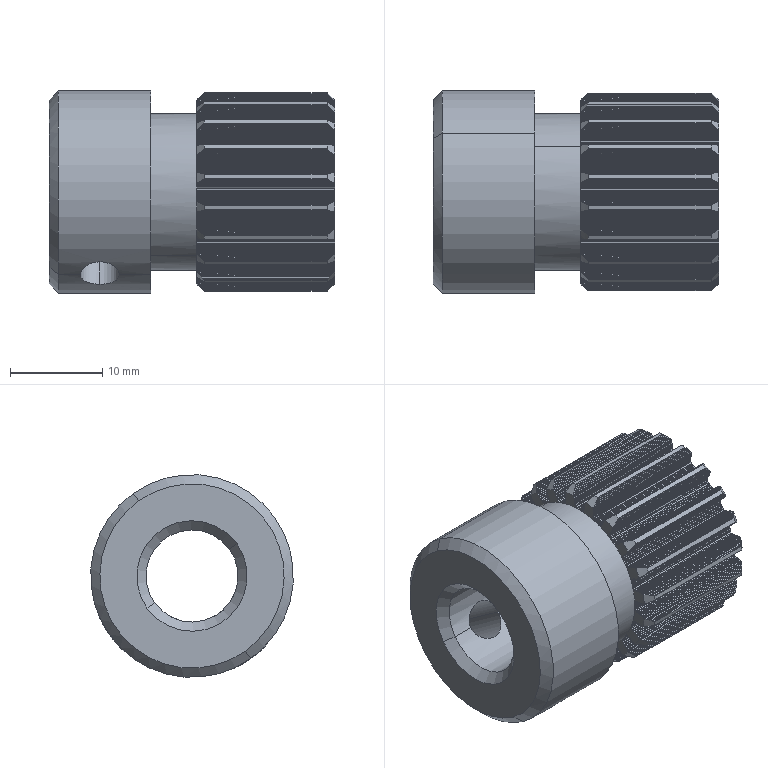Component | SolidWorks | FilmMechanism-3-1_Gear-1 | 1 solid | 1299 faces | volume 6893 mm3 | plane 1243 | cone 46 | cylinder 10 | commonest cylinder face diameters 4.2 x4 10 x2 22 x2 17 x2